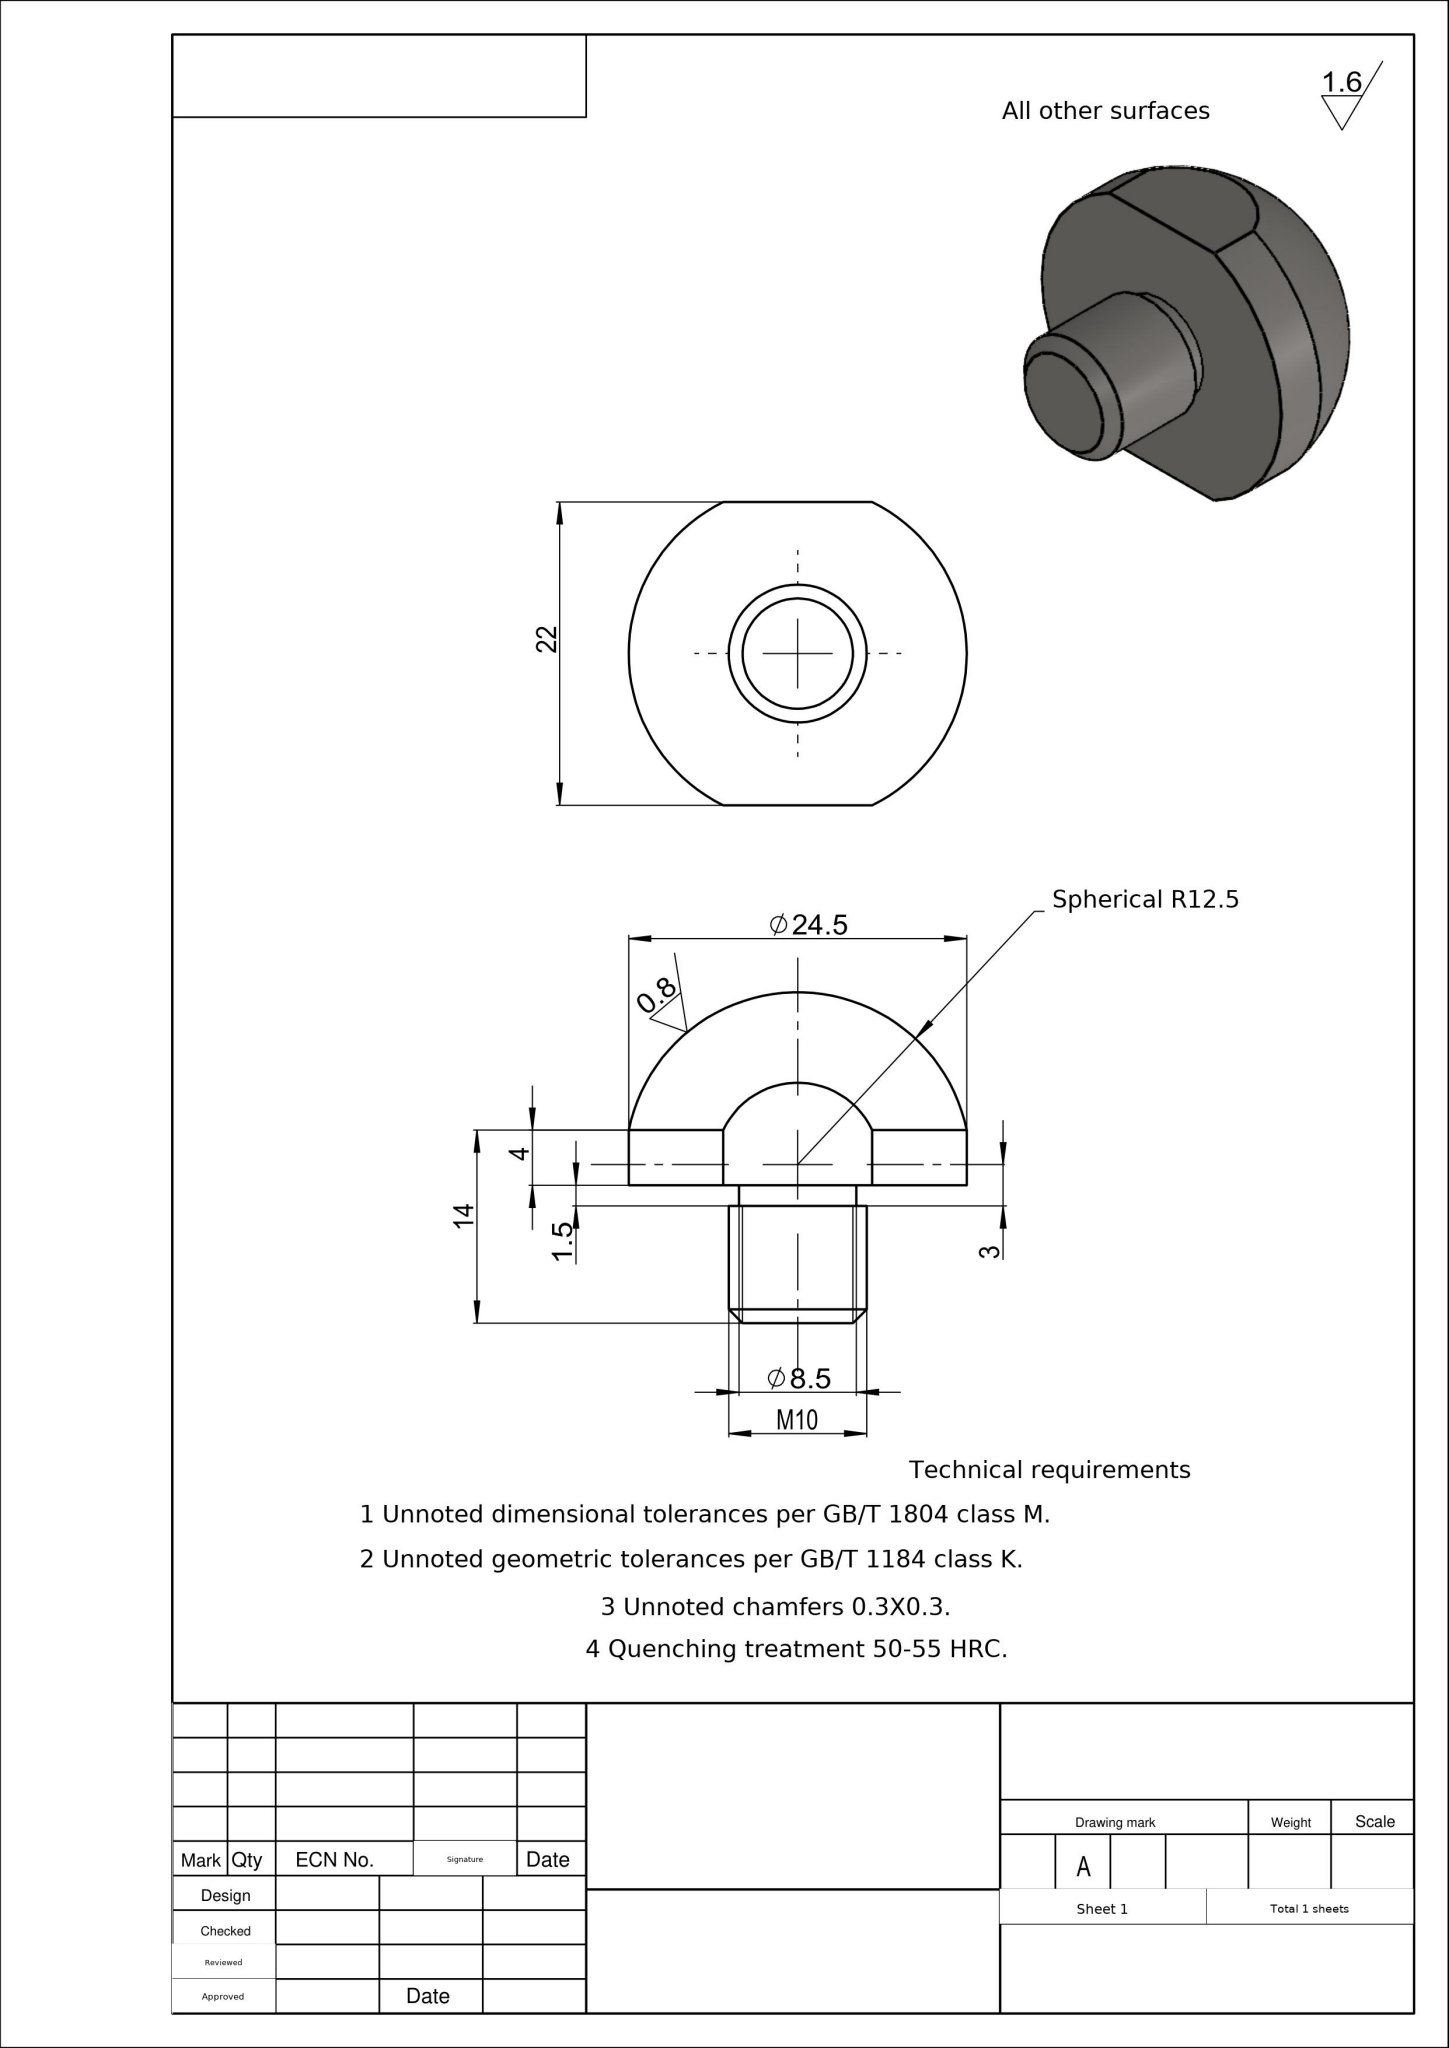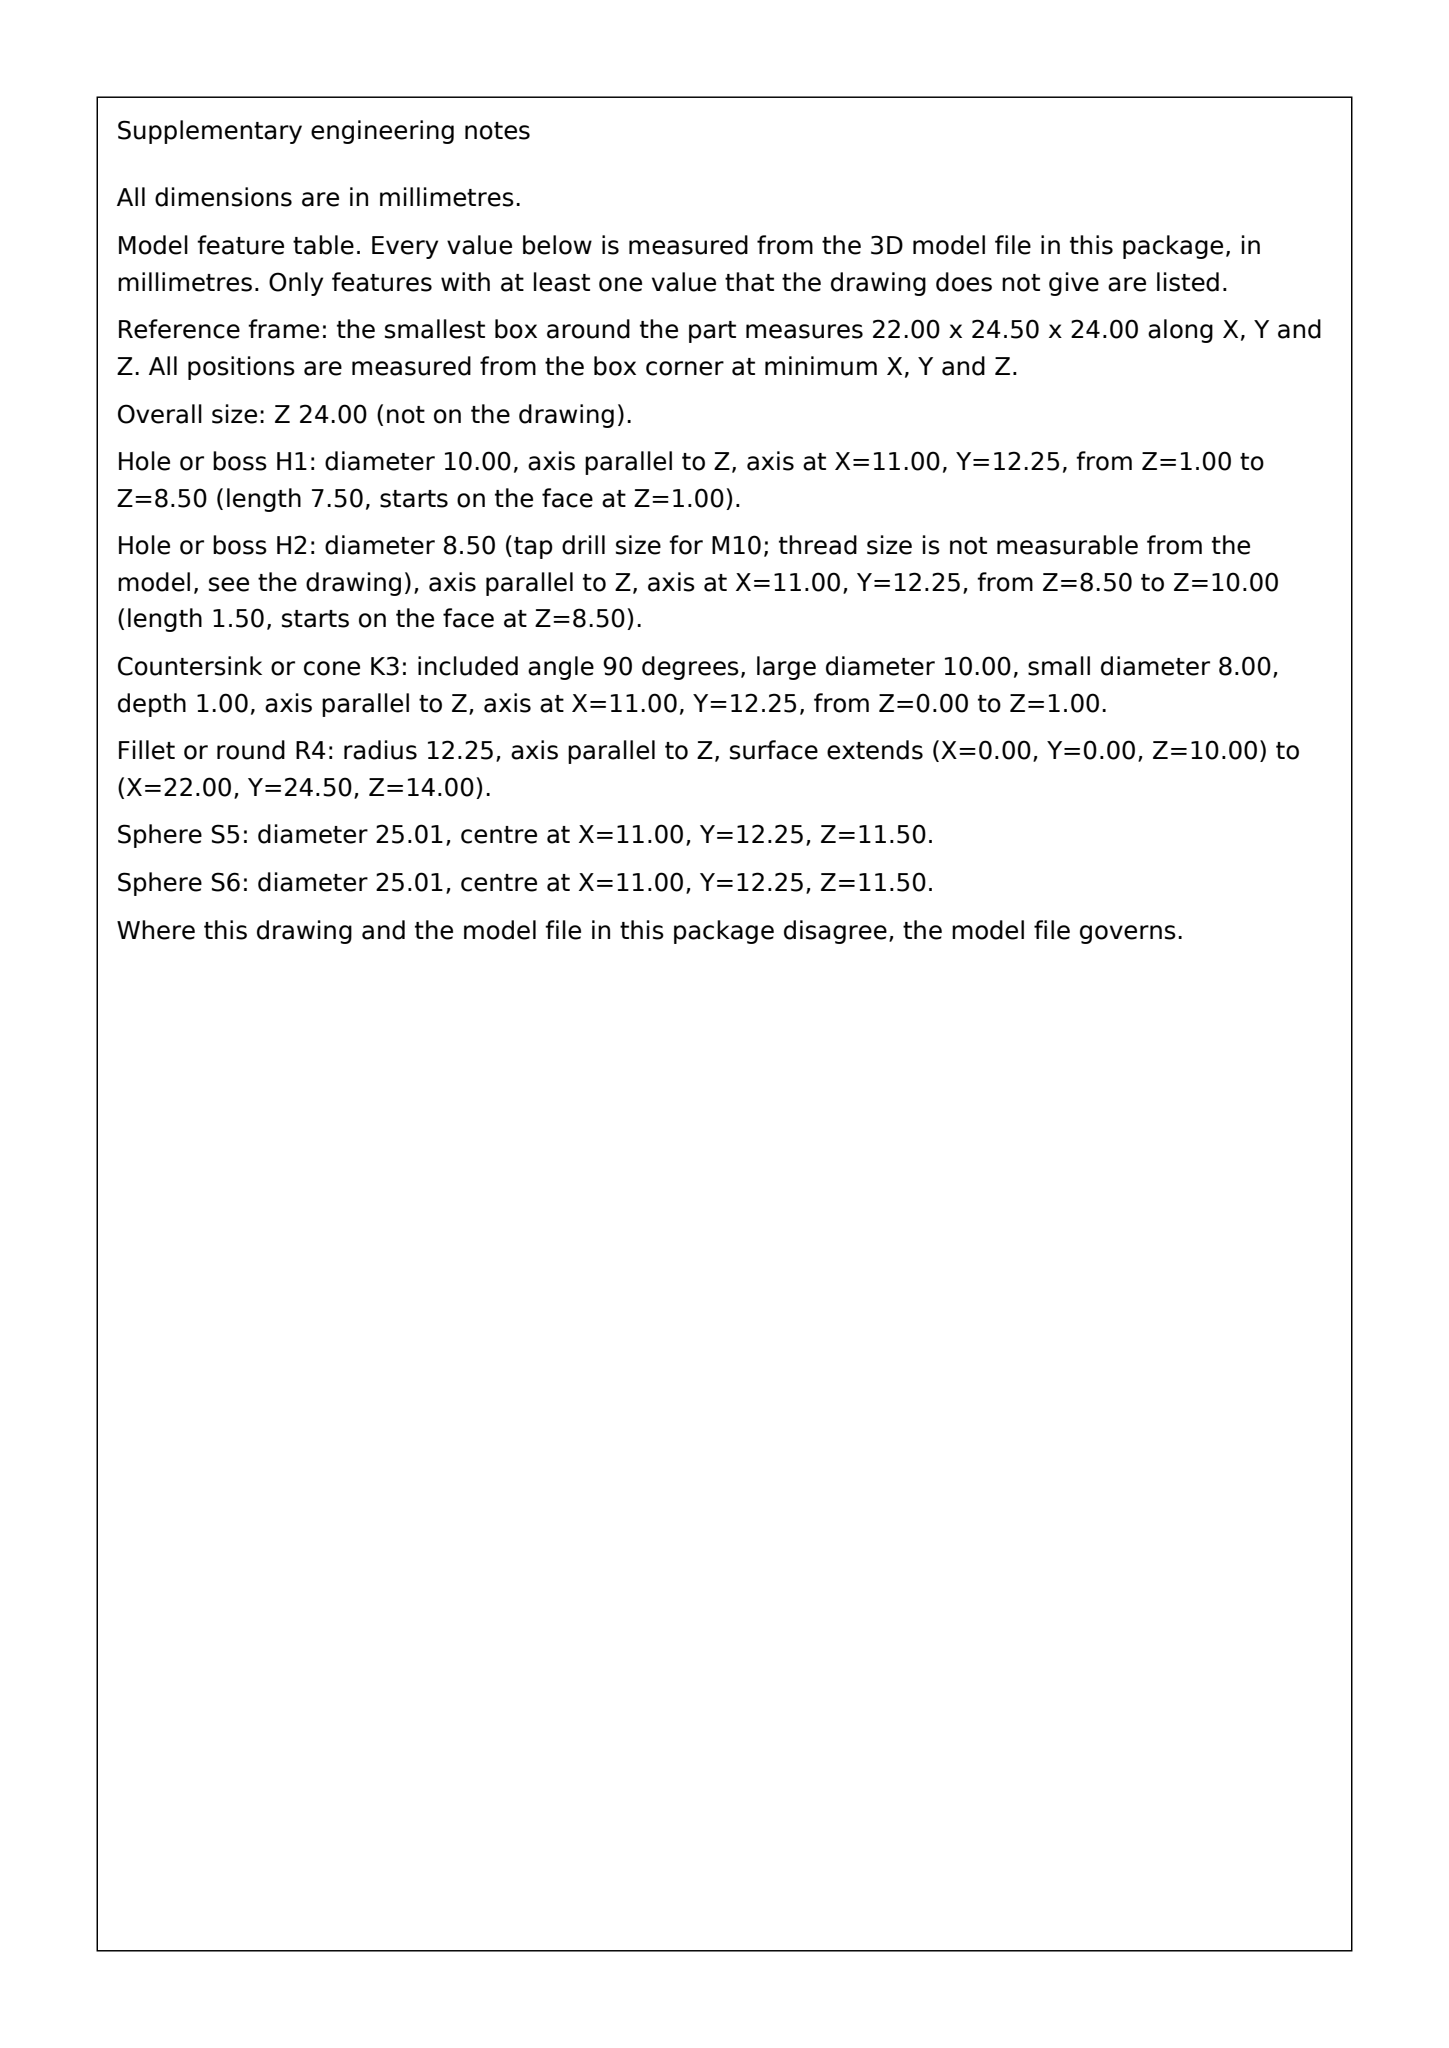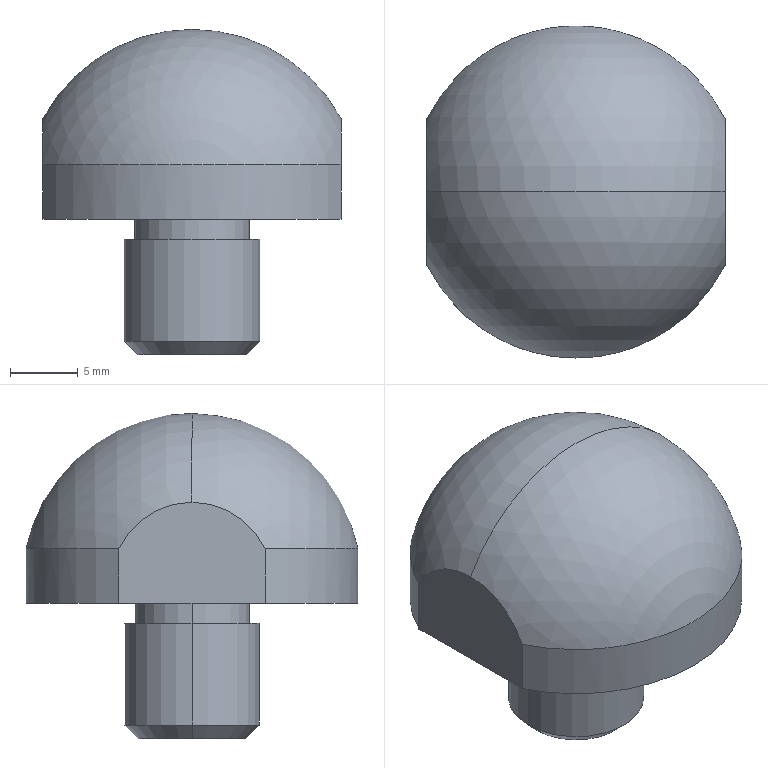Part | SolidWorks | mm | 1 solid | 15 faces | box 22 x 24.5 x 24 mm | volume 5402 mm3 | cylinder 6 | plane 5 | cone 2 | sphere 2 | commonest cylinder face diameters 10 x2 8.5 x2 24.5 x2
build123d program:
from build123d import *

# Parameters (mm, degrees)
SKETCH1_R           = 5
BOSS_EXTRUDE1_DEPTH = 10
SKETCH2_R           = 12.25
BOSS_EXTRUDE2_DEPTH = 4
DOME1_FACE_RADIUS   = 12.25
DOME1_HEIGHT        = 10
SKETCH3_OUTSIDE_W   = 34.93
SKETCH3_OUTSIDE_H   = 34.93
SKETCH3_OUTSIDE_R   = 4.25
CUT_EXTRUDE1_DEPTH  = 1.5
CHAMFER1_SIZE       = 1
SKETCH4_OUTSIDE_W   = 34.93
SKETCH4_OUTSIDE_H   = 34.93
SKETCH4_OUTSIDE_W_2 = 22
SKETCH4_OUTSIDE_H_2 = 31.445
CUT_EXTRUDE3_DEPTH  = 30.599


with BuildPart() as part:
    # Sketch1 → Boss-Extrude1 (new body)
    with BuildSketch(Plane.XY):
        Circle(SKETCH1_R)
    extrude(amount=BOSS_EXTRUDE1_DEPTH)

    # Sketch2 → Boss-Extrude2 (add)
    with BuildSketch(Plane.XY.offset(10)):
        Circle(SKETCH2_R)
    extrude(amount=BOSS_EXTRUDE2_DEPTH)

    # Dome1: a dome of height H over a round flat face of radius A is a cap of a sphere of radius (A * A + H * H) / (2 * H)
    dome1_r = (DOME1_FACE_RADIUS * DOME1_FACE_RADIUS + DOME1_HEIGHT * DOME1_HEIGHT) / (2 * DOME1_HEIGHT)
    dome1_base = Plane((0, 0, 14), z_dir=(0, 0, 1))
    with Locations(dome1_base.offset(DOME1_HEIGHT - dome1_r)):
        dome1_ball = Sphere(dome1_r, mode=Mode.PRIVATE)
    add(split(dome1_ball, bisect_by=dome1_base, keep=Keep.TOP, mode=Mode.PRIVATE))

    # Sketch3 outside → Cut-Extrude1 (cut)
    with BuildSketch(Plane(origin=(0, 0, 10), x_dir=(-1, 0, 0), z_dir=(0, 0, -1))):
        Rectangle(SKETCH3_OUTSIDE_W, SKETCH3_OUTSIDE_H)
        Circle(SKETCH3_OUTSIDE_R, mode=Mode.SUBTRACT)
    extrude(amount=CUT_EXTRUDE1_DEPTH, mode=Mode.SUBTRACT)

    # Chamfer1
    chamfer1_edges = [part.edges().sort_by_distance(p)[0] for p in [
        (-5, 0, 0),
    ]]
    chamfer(chamfer1_edges, length=CHAMFER1_SIZE)

    # Sketch4 outside → Cut-Extrude3 (cut, through all)
    with BuildSketch(Plane.XY):
        Rectangle(SKETCH4_OUTSIDE_W, SKETCH4_OUTSIDE_H)
        with Locations((0, -0.3628)):
            Rectangle(SKETCH4_OUTSIDE_W_2, SKETCH4_OUTSIDE_H_2, mode=Mode.SUBTRACT)
    extrude(amount=CUT_EXTRUDE3_DEPTH, mode=Mode.SUBTRACT)


solid = part.part
STEP:
#1=CARTESIAN_POINT('',(-4.,0.,0.));
#2=VERTEX_POINT('',#1);
#3=CARTESIAN_POINT('',(4.,0.,0.));
#4=VERTEX_POINT('',#3);
#5=CARTESIAN_POINT('',(0.,0.,0.));
#6=DIRECTION('',(0.,0.,-1.));
#7=DIRECTION('',(1.,0.,0.));
#8=AXIS2_PLACEMENT_3D('',#5,#6,#7);
#9=CIRCLE('',#8,4.);
#10=EDGE_CURVE('',#2,#4,#9,.T.);
#11=ORIENTED_EDGE('',*,*,#10,.F.);
#12=CARTESIAN_POINT('',(-5.,0.,1.));
#13=VERTEX_POINT('',#12);
#14=CARTESIAN_POINT('',(-5.,0.,1.));
#15=DIRECTION('',(-0.7071,0.,0.7071));
#16=VECTOR('',#15,1000.);
#17=LINE('',#14,#16);
#18=EDGE_CURVE('',#2,#13,#17,.T.);
#19=ORIENTED_EDGE('',*,*,#18,.T.);
#20=CARTESIAN_POINT('',(5.,0.,1.));
#21=VERTEX_POINT('',#20);
#22=CARTESIAN_POINT('',(0.,0.,1.));
#23=DIRECTION('',(0.,0.,1.));
#24=DIRECTION('',(1.,0.,0.));
#25=AXIS2_PLACEMENT_3D('',#22,#23,#24);
#26=CIRCLE('',#25,5.);
#27=EDGE_CURVE('',#21,#13,#26,.T.);
#28=ORIENTED_EDGE('',*,*,#27,.F.);
#29=CARTESIAN_POINT('',(5.,0.,1.));
#30=DIRECTION('',(0.7071,0.,0.7071));
#31=VECTOR('',#30,1000.);
#32=LINE('',#29,#31);
#33=EDGE_CURVE('',#4,#21,#32,.T.);
#34=ORIENTED_EDGE('',*,*,#33,.F.);
#35=EDGE_LOOP('',(#11,#19,#28,#34));
#36=FACE_OUTER_BOUND('',#35,.T.);
#37=CARTESIAN_POINT('',(0.,0.,1.));
#38=DIRECTION('',(0.,0.,1.));
#39=DIRECTION('',(1.,0.,0.));
#40=AXIS2_PLACEMENT_3D('',#37,#38,#39);
#41=CONICAL_SURFACE('',#40,5.,0.7854);
#42=ADVANCED_FACE('',(#36),#41,.T.);
#43=CARTESIAN_POINT('',(-5.,0.,8.5));
#44=VERTEX_POINT('',#43);
#45=CARTESIAN_POINT('',(5.,0.,8.5));
#46=VERTEX_POINT('',#45);
#47=CARTESIAN_POINT('',(0.,0.,8.5));
#48=DIRECTION('',(0.,0.,-1.));
#49=DIRECTION('',(-1.,0.,0.));
#50=AXIS2_PLACEMENT_3D('',#47,#48,#49);
#51=CIRCLE('',#50,5.);
#52=EDGE_CURVE('',#44,#46,#51,.T.);
#53=ORIENTED_EDGE('',*,*,#52,.T.);
#54=CARTESIAN_POINT('',(5.,0.,10.));
#55=DIRECTION('',(0.,0.,-1.));
#56=VECTOR('',#55,1000.);
#57=LINE('',#54,#56);
#58=EDGE_CURVE('',#46,#21,#57,.T.);
#59=ORIENTED_EDGE('',*,*,#58,.T.);
#60=ORIENTED_EDGE('',*,*,#27,.T.);
#61=CARTESIAN_POINT('',(-5.,0.,10.));
#62=DIRECTION('',(0.,0.,-1.));
#63=VECTOR('',#62,1000.);
#64=LINE('',#61,#63);
#65=EDGE_CURVE('',#44,#13,#64,.T.);
#66=ORIENTED_EDGE('',*,*,#65,.F.);
#67=EDGE_LOOP('',(#53,#59,#60,#66));
#68=FACE_OUTER_BOUND('',#67,.T.);
#69=CARTESIAN_POINT('',(0.,0.,10.));
#70=DIRECTION('',(0.,0.,-1.));
#71=DIRECTION('',(-1.,0.,0.));
#72=AXIS2_PLACEMENT_3D('',#69,#70,#71);
#73=CYLINDRICAL_SURFACE('',#72,5.);
#74=ADVANCED_FACE('',(#68),#73,.T.);
#75=CARTESIAN_POINT('',(-4.25,0.,8.5));
#76=VERTEX_POINT('',#75);
#77=CARTESIAN_POINT('',(4.25,0.,8.5));
#78=VERTEX_POINT('',#77);
#79=CARTESIAN_POINT('',(0.,0.,8.5));
#80=DIRECTION('',(0.,0.,-1.));
#81=DIRECTION('',(-1.,0.,0.));
#82=AXIS2_PLACEMENT_3D('',#79,#80,#81);
#83=CIRCLE('',#82,4.25);
#84=EDGE_CURVE('',#76,#78,#83,.T.);
#85=ORIENTED_EDGE('',*,*,#84,.F.);
#86=CARTESIAN_POINT('',(-4.25,0.,10.));
#87=VERTEX_POINT('',#86);
#88=CARTESIAN_POINT('',(-4.25,0.,8.5));
#89=DIRECTION('',(0.,0.,1.));
#90=VECTOR('',#89,1000.);
#91=LINE('',#88,#90);
#92=EDGE_CURVE('',#76,#87,#91,.T.);
#93=ORIENTED_EDGE('',*,*,#92,.T.);
#94=CARTESIAN_POINT('',(4.25,0.,10.));
#95=VERTEX_POINT('',#94);
#96=CARTESIAN_POINT('',(0.,0.,10.));
#97=DIRECTION('',(0.,0.,-1.));
#98=DIRECTION('',(-1.,0.,0.));
#99=AXIS2_PLACEMENT_3D('',#96,#97,#98);
#100=CIRCLE('',#99,4.25);
#101=EDGE_CURVE('',#87,#95,#100,.T.);
#102=ORIENTED_EDGE('',*,*,#101,.T.);
#103=CARTESIAN_POINT('',(4.25,0.,8.5));
#104=DIRECTION('',(0.,0.,1.));
#105=VECTOR('',#104,1000.);
#106=LINE('',#103,#105);
#107=EDGE_CURVE('',#78,#95,#106,.T.);
#108=ORIENTED_EDGE('',*,*,#107,.F.);
#109=EDGE_LOOP('',(#85,#93,#102,#108));
#110=FACE_OUTER_BOUND('',#109,.T.);
#111=CARTESIAN_POINT('',(0.,0.,8.5));
#112=DIRECTION('',(0.,0.,1.));
#113=DIRECTION('',(1.,0.,0.));
#114=AXIS2_PLACEMENT_3D('',#111,#112,#113);
#115=CYLINDRICAL_SURFACE('',#114,4.25);
#116=ADVANCED_FACE('',(#110),#115,.T.);
#117=CARTESIAN_POINT('',(-11.,0.,17.441));
#118=VERTEX_POINT('',#117);
#119=CARTESIAN_POINT('',(-11.,5.391,14.));
#120=VERTEX_POINT('',#119);
#121=CARTESIAN_POINT('',(-11.,-0.,11.497));
#122=DIRECTION('',(-1.,-0.,0.));
#123=DIRECTION('',(0.,1.,-0.));
#124=AXIS2_PLACEMENT_3D('',#121,#122,#123);
#125=CIRCLE('',#124,5.944);
#126=EDGE_CURVE('',#118,#120,#125,.T.);
#127=ORIENTED_EDGE('',*,*,#126,.F.);
#128=CARTESIAN_POINT('',(0.,0.,24.));
#129=VERTEX_POINT('',#128);
#130=CARTESIAN_POINT('',(0.,0.,11.497));
#131=DIRECTION('',(0.,1.,0.));
#132=DIRECTION('',(-1.,0.,0.));
#133=AXIS2_PLACEMENT_3D('',#130,#131,#132);
#134=CIRCLE('',#133,12.503);
#135=EDGE_CURVE('',#118,#129,#134,.T.);
#136=ORIENTED_EDGE('',*,*,#135,.T.);
#137=CARTESIAN_POINT('',(11.,0.,17.441));
#138=VERTEX_POINT('',#137);
#139=CARTESIAN_POINT('',(0.,0.,11.497));
#140=DIRECTION('',(0.,-1.,0.));
#141=DIRECTION('',(0.,0.,-1.));
#142=AXIS2_PLACEMENT_3D('',#139,#140,#141);
#143=CIRCLE('',#142,12.503);
#144=EDGE_CURVE('',#138,#129,#143,.T.);
#145=ORIENTED_EDGE('',*,*,#144,.F.);
#146=CARTESIAN_POINT('',(11.,5.391,14.));
#147=VERTEX_POINT('',#146);
#148=CARTESIAN_POINT('',(11.,0.,11.497));
#149=DIRECTION('',(1.,0.,0.));
#150=DIRECTION('',(0.,-1.,0.));
#151=AXIS2_PLACEMENT_3D('',#148,#149,#150);
#152=CIRCLE('',#151,5.944);
#153=EDGE_CURVE('',#147,#138,#152,.T.);
#154=ORIENTED_EDGE('',*,*,#153,.F.);
#155=CARTESIAN_POINT('',(0.,0.,14.));
#156=DIRECTION('',(0.,0.,1.));
#157=DIRECTION('',(1.,0.,0.));
#158=AXIS2_PLACEMENT_3D('',#155,#156,#157);
#159=CIRCLE('',#158,12.25);
#160=EDGE_CURVE('',#147,#120,#159,.T.);
#161=ORIENTED_EDGE('',*,*,#160,.T.);
#162=EDGE_LOOP('',(#127,#136,#145,#154,#161));
#163=FACE_OUTER_BOUND('',#162,.T.);
#164=CARTESIAN_POINT('',(0.,0.,11.497));
#165=DIRECTION('',(0.,1.,0.));
#166=DIRECTION('',(1.,0.,0.));
#167=AXIS2_PLACEMENT_3D('',#164,#165,#166);
#168=SPHERICAL_SURFACE('',#167,12.503);
#169=ADVANCED_FACE('',(#163),#168,.T.);
#170=CARTESIAN_POINT('',(-11.,-5.391,14.));
#171=VERTEX_POINT('',#170);
#172=CARTESIAN_POINT('',(11.,-5.391,14.));
#173=VERTEX_POINT('',#172);
#174=CARTESIAN_POINT('',(0.,0.,14.));
#175=DIRECTION('',(0.,0.,1.));
#176=DIRECTION('',(1.,0.,0.));
#177=AXIS2_PLACEMENT_3D('',#174,#175,#176);
#178=CIRCLE('',#177,12.25);
#179=EDGE_CURVE('',#171,#173,#178,.T.);
#180=ORIENTED_EDGE('',*,*,#179,.F.);
#181=CARTESIAN_POINT('',(-11.,-5.391,10.));
#182=VERTEX_POINT('',#181);
#183=CARTESIAN_POINT('',(-11.,-5.391,14.));
#184=DIRECTION('',(0.,0.,-1.));
#185=VECTOR('',#184,1000.);
#186=LINE('',#183,#185);
#187=EDGE_CURVE('',#171,#182,#186,.T.);
#188=ORIENTED_EDGE('',*,*,#187,.T.);
#189=CARTESIAN_POINT('',(11.,-5.391,10.));
#190=VERTEX_POINT('',#189);
#191=CARTESIAN_POINT('',(0.,0.,10.));
#192=DIRECTION('',(0.,0.,1.));
#193=DIRECTION('',(1.,0.,0.));
#194=AXIS2_PLACEMENT_3D('',#191,#192,#193);
#195=CIRCLE('',#194,12.25);
#196=EDGE_CURVE('',#182,#190,#195,.T.);
#197=ORIENTED_EDGE('',*,*,#196,.T.);
#198=CARTESIAN_POINT('',(11.,-5.391,14.));
#199=DIRECTION('',(0.,0.,1.));
#200=VECTOR('',#199,1000.);
#201=LINE('',#198,#200);
#202=EDGE_CURVE('',#190,#173,#201,.T.);
#203=ORIENTED_EDGE('',*,*,#202,.T.);
#204=EDGE_LOOP('',(#180,#188,#197,#203));
#205=FACE_OUTER_BOUND('',#204,.T.);
#206=CARTESIAN_POINT('',(0.,0.,14.));
#207=DIRECTION('',(0.,0.,-1.));
#208=DIRECTION('',(-1.,0.,0.));
#209=AXIS2_PLACEMENT_3D('',#206,#207,#208);
#210=CYLINDRICAL_SURFACE('',#209,12.25);
#211=ADVANCED_FACE('',(#205),#210,.T.);
#212=ORIENTED_EDGE('',*,*,#196,.F.);
#213=CARTESIAN_POINT('',(-11.,5.391,10.));
#214=VERTEX_POINT('',#213);
#215=CARTESIAN_POINT('',(-11.,-0.,10.));
#216=DIRECTION('',(-0.,1.,0.));
#217=VECTOR('',#216,1000.);
#218=LINE('',#215,#217);
#219=EDGE_CURVE('',#182,#214,#218,.T.);
#220=ORIENTED_EDGE('',*,*,#219,.T.);
#221=CARTESIAN_POINT('',(11.,5.391,10.));
#222=VERTEX_POINT('',#221);
#223=CARTESIAN_POINT('',(0.,0.,10.));
#224=DIRECTION('',(0.,0.,1.));
#225=DIRECTION('',(1.,0.,0.));
#226=AXIS2_PLACEMENT_3D('',#223,#224,#225);
#227=CIRCLE('',#226,12.25);
#228=EDGE_CURVE('',#222,#214,#227,.T.);
#229=ORIENTED_EDGE('',*,*,#228,.F.);
#230=CARTESIAN_POINT('',(11.,0.,10.));
#231=DIRECTION('',(0.,-1.,0.));
#232=VECTOR('',#231,1000.);
#233=LINE('',#230,#232);
#234=EDGE_CURVE('',#222,#190,#233,.T.);
#235=ORIENTED_EDGE('',*,*,#234,.T.);
#236=EDGE_LOOP('',(#212,#220,#229,#235));
#237=FACE_OUTER_BOUND('',#236,.T.);
#238=CARTESIAN_POINT('',(0.,0.,10.));
#239=DIRECTION('',(0.,0.,-1.));
#240=DIRECTION('',(-1.,0.,0.));
#241=AXIS2_PLACEMENT_3D('',#238,#239,#240);
#242=CIRCLE('',#241,4.25);
#243=EDGE_CURVE('',#95,#87,#242,.T.);
#244=ORIENTED_EDGE('',*,*,#243,.F.);
#245=ORIENTED_EDGE('',*,*,#101,.F.);
#246=EDGE_LOOP('',(#244,#245));
#247=FACE_BOUND('',#246,.T.);
#248=CARTESIAN_POINT('',(0.,0.,10.));
#249=DIRECTION('',(0.,0.,1.));
#250=DIRECTION('',(1.,0.,0.));
#251=AXIS2_PLACEMENT_3D('',#248,#249,#250);
#252=PLANE('',#251);
#253=ADVANCED_FACE('',(#237,#247),#252,.F.);
#254=ORIENTED_EDGE('',*,*,#228,.T.);
#255=CARTESIAN_POINT('',(-11.,5.391,14.));
#256=DIRECTION('',(0.,0.,1.));
#257=VECTOR('',#256,1000.);
#258=LINE('',#255,#257);
#259=EDGE_CURVE('',#214,#120,#258,.T.);
#260=ORIENTED_EDGE('',*,*,#259,.T.);
#261=ORIENTED_EDGE('',*,*,#160,.F.);
#262=CARTESIAN_POINT('',(11.,5.391,14.));
#263=DIRECTION('',(0.,0.,-1.));
#264=VECTOR('',#263,1000.);
#265=LINE('',#262,#264);
#266=EDGE_CURVE('',#147,#222,#265,.T.);
#267=ORIENTED_EDGE('',*,*,#266,.T.);
#268=EDGE_LOOP('',(#254,#260,#261,#267));
#269=FACE_OUTER_BOUND('',#268,.T.);
#270=CARTESIAN_POINT('',(0.,0.,14.));
#271=DIRECTION('',(0.,0.,-1.));
#272=DIRECTION('',(-1.,0.,0.));
#273=AXIS2_PLACEMENT_3D('',#270,#271,#272);
#274=CYLINDRICAL_SURFACE('',#273,12.25);
#275=ADVANCED_FACE('',(#269),#274,.T.);
#276=ORIENTED_EDGE('',*,*,#135,.F.);
#277=CARTESIAN_POINT('',(-11.,-0.,11.497));
#278=DIRECTION('',(-1.,-0.,0.));
#279=DIRECTION('',(0.,1.,0.));
#280=AXIS2_PLACEMENT_3D('',#277,#278,#279);
#281=CIRCLE('',#280,5.944);
#282=EDGE_CURVE('',#171,#118,#281,.T.);
#283=ORIENTED_EDGE('',*,*,#282,.F.);
#284=ORIENTED_EDGE('',*,*,#179,.T.);
#285=CARTESIAN_POINT('',(11.,0.,11.497));
#286=DIRECTION('',(1.,0.,0.));
#287=DIRECTION('',(0.,-1.,0.));
#288=AXIS2_PLACEMENT_3D('',#285,#286,#287);
#289=CIRCLE('',#288,5.944);
#290=EDGE_CURVE('',#138,#173,#289,.T.);
#291=ORIENTED_EDGE('',*,*,#290,.F.);
#292=ORIENTED_EDGE('',*,*,#144,.T.);
#293=EDGE_LOOP('',(#276,#283,#284,#291,#292));
#294=FACE_OUTER_BOUND('',#293,.T.);
#295=CARTESIAN_POINT('',(0.,0.,11.497));
#296=DIRECTION('',(0.,1.,0.));
#297=DIRECTION('',(1.,0.,0.));
#298=AXIS2_PLACEMENT_3D('',#295,#296,#297);
#299=SPHERICAL_SURFACE('',#298,12.503);
#300=ADVANCED_FACE('',(#294),#299,.T.);
#301=CARTESIAN_POINT('',(0.,0.,8.5));
#302=DIRECTION('',(0.,0.,-1.));
#303=DIRECTION('',(-1.,0.,0.));
#304=AXIS2_PLACEMENT_3D('',#301,#302,#303);
#305=CIRCLE('',#304,4.25);
#306=EDGE_CURVE('',#78,#76,#305,.T.);
#307=ORIENTED_EDGE('',*,*,#306,.T.);
#308=ORIENTED_EDGE('',*,*,#84,.T.);
#309=EDGE_LOOP('',(#307,#308));
#310=FACE_BOUND('',#309,.T.);
#311=ORIENTED_EDGE('',*,*,#52,.F.);
#312=CARTESIAN_POINT('',(0.,0.,8.5));
#313=DIRECTION('',(0.,0.,-1.));
#314=DIRECTION('',(-1.,0.,0.));
#315=AXIS2_PLACEMENT_3D('',#312,#313,#314);
#316=CIRCLE('',#315,5.);
#317=EDGE_CURVE('',#46,#44,#316,.T.);
#318=ORIENTED_EDGE('',*,*,#317,.F.);
#319=EDGE_LOOP('',(#311,#318));
#320=FACE_OUTER_BOUND('',#319,.T.);
#321=CARTESIAN_POINT('',(0.,0.,8.5));
#322=DIRECTION('',(0.,0.,-1.));
#323=DIRECTION('',(-1.,0.,0.));
#324=AXIS2_PLACEMENT_3D('',#321,#322,#323);
#325=PLANE('',#324);
#326=ADVANCED_FACE('',(#310,#320),#325,.F.);
#327=ORIENTED_EDGE('',*,*,#92,.F.);
#328=ORIENTED_EDGE('',*,*,#306,.F.);
#329=ORIENTED_EDGE('',*,*,#107,.T.);
#330=ORIENTED_EDGE('',*,*,#243,.T.);
#331=EDGE_LOOP('',(#327,#328,#329,#330));
#332=FACE_OUTER_BOUND('',#331,.T.);
#333=CARTESIAN_POINT('',(0.,0.,8.5));
#334=DIRECTION('',(0.,0.,1.));
#335=DIRECTION('',(1.,0.,0.));
#336=AXIS2_PLACEMENT_3D('',#333,#334,#335);
#337=CYLINDRICAL_SURFACE('',#336,4.25);
#338=ADVANCED_FACE('',(#332),#337,.T.);
#339=CARTESIAN_POINT('',(0.,0.,0.));
#340=DIRECTION('',(0.,0.,-1.));
#341=DIRECTION('',(1.,0.,0.));
#342=AXIS2_PLACEMENT_3D('',#339,#340,#341);
#343=CIRCLE('',#342,4.);
#344=EDGE_CURVE('',#4,#2,#343,.T.);
#345=ORIENTED_EDGE('',*,*,#344,.T.);
#346=ORIENTED_EDGE('',*,*,#10,.T.);
#347=EDGE_LOOP('',(#345,#346));
#348=FACE_OUTER_BOUND('',#347,.T.);
#349=CARTESIAN_POINT('',(0.,0.,0.));
#350=DIRECTION('',(0.,0.,1.));
#351=DIRECTION('',(1.,0.,0.));
#352=AXIS2_PLACEMENT_3D('',#349,#350,#351);
#353=PLANE('',#352);
#354=ADVANCED_FACE('',(#348),#353,.F.);
#355=ORIENTED_EDGE('',*,*,#58,.F.);
#356=ORIENTED_EDGE('',*,*,#317,.T.);
#357=ORIENTED_EDGE('',*,*,#65,.T.);
#358=CARTESIAN_POINT('',(0.,0.,1.));
#359=DIRECTION('',(0.,0.,1.));
#360=DIRECTION('',(1.,0.,0.));
#361=AXIS2_PLACEMENT_3D('',#358,#359,#360);
#362=CIRCLE('',#361,5.);
#363=EDGE_CURVE('',#13,#21,#362,.T.);
#364=ORIENTED_EDGE('',*,*,#363,.T.);
#365=EDGE_LOOP('',(#355,#356,#357,#364));
#366=FACE_OUTER_BOUND('',#365,.T.);
#367=CARTESIAN_POINT('',(0.,0.,10.));
#368=DIRECTION('',(0.,0.,-1.));
#369=DIRECTION('',(-1.,0.,0.));
#370=AXIS2_PLACEMENT_3D('',#367,#368,#369);
#371=CYLINDRICAL_SURFACE('',#370,5.);
#372=ADVANCED_FACE('',(#366),#371,.T.);
#373=ORIENTED_EDGE('',*,*,#18,.F.);
#374=ORIENTED_EDGE('',*,*,#344,.F.);
#375=ORIENTED_EDGE('',*,*,#33,.T.);
#376=ORIENTED_EDGE('',*,*,#363,.F.);
#377=EDGE_LOOP('',(#373,#374,#375,#376));
#378=FACE_OUTER_BOUND('',#377,.T.);
#379=CARTESIAN_POINT('',(0.,0.,1.));
#380=DIRECTION('',(0.,0.,1.));
#381=DIRECTION('',(1.,0.,0.));
#382=AXIS2_PLACEMENT_3D('',#379,#380,#381);
#383=CONICAL_SURFACE('',#382,5.,0.7854);
#384=ADVANCED_FACE('',(#378),#383,.T.);
#385=ORIENTED_EDGE('',*,*,#266,.F.);
#386=ORIENTED_EDGE('',*,*,#153,.T.);
#387=ORIENTED_EDGE('',*,*,#290,.T.);
#388=ORIENTED_EDGE('',*,*,#202,.F.);
#389=ORIENTED_EDGE('',*,*,#234,.F.);
#390=EDGE_LOOP('',(#385,#386,#387,#388,#389));
#391=FACE_OUTER_BOUND('',#390,.T.);
#392=CARTESIAN_POINT('',(11.,15.36,24.));
#393=DIRECTION('',(-1.,-0.,0.));
#394=DIRECTION('',(0.,-1.,0.));
#395=AXIS2_PLACEMENT_3D('',#392,#393,#394);
#396=PLANE('',#395);
#397=ADVANCED_FACE('',(#391),#396,.F.);
#398=ORIENTED_EDGE('',*,*,#187,.F.);
#399=ORIENTED_EDGE('',*,*,#282,.T.);
#400=ORIENTED_EDGE('',*,*,#126,.T.);
#401=ORIENTED_EDGE('',*,*,#259,.F.);
#402=ORIENTED_EDGE('',*,*,#219,.F.);
#403=EDGE_LOOP('',(#398,#399,#400,#401,#402));
#404=FACE_OUTER_BOUND('',#403,.T.);
#405=CARTESIAN_POINT('',(-11.,15.36,24.));
#406=DIRECTION('',(1.,0.,0.));
#407=DIRECTION('',(-0.,1.,0.));
#408=AXIS2_PLACEMENT_3D('',#405,#406,#407);
#409=PLANE('',#408);
#410=ADVANCED_FACE('',(#404),#409,.F.);
#411=CLOSED_SHELL('',(#42,#74,#116,#169,#211,#253,#275,#300,#326,#338,#354,#372,#384,#397,#410));
#412=MANIFOLD_SOLID_BREP('',#411);
#413=CARTESIAN_POINT('',(0.,0.,0.));
#414=DIRECTION('',(0.,0.,1.));
#415=DIRECTION('',(1.,0.,0.));
#416=AXIS2_PLACEMENT_3D('',#413,#414,#415);
#417=(LENGTH_UNIT()NAMED_UNIT(*)SI_UNIT(.MILLI.,.METRE.));
#418=UNCERTAINTY_MEASURE_WITH_UNIT(LENGTH_MEASURE(0.00001),#417,'','');
#419=(NAMED_UNIT(*)PLANE_ANGLE_UNIT()SI_UNIT($,.RADIAN.));
#420=(NAMED_UNIT(*)SI_UNIT($,.STERADIAN.)SOLID_ANGLE_UNIT());
#421=(GEOMETRIC_REPRESENTATION_CONTEXT(3)GLOBAL_UNCERTAINTY_ASSIGNED_CONTEXT((#418))GLOBAL_UNIT_ASSIGNED_CONTEXT((#417,#419,#420))REPRESENTATION_CONTEXT('',''));
#422=ADVANCED_BREP_SHAPE_REPRESENTATION('',(#412,#416),#421);